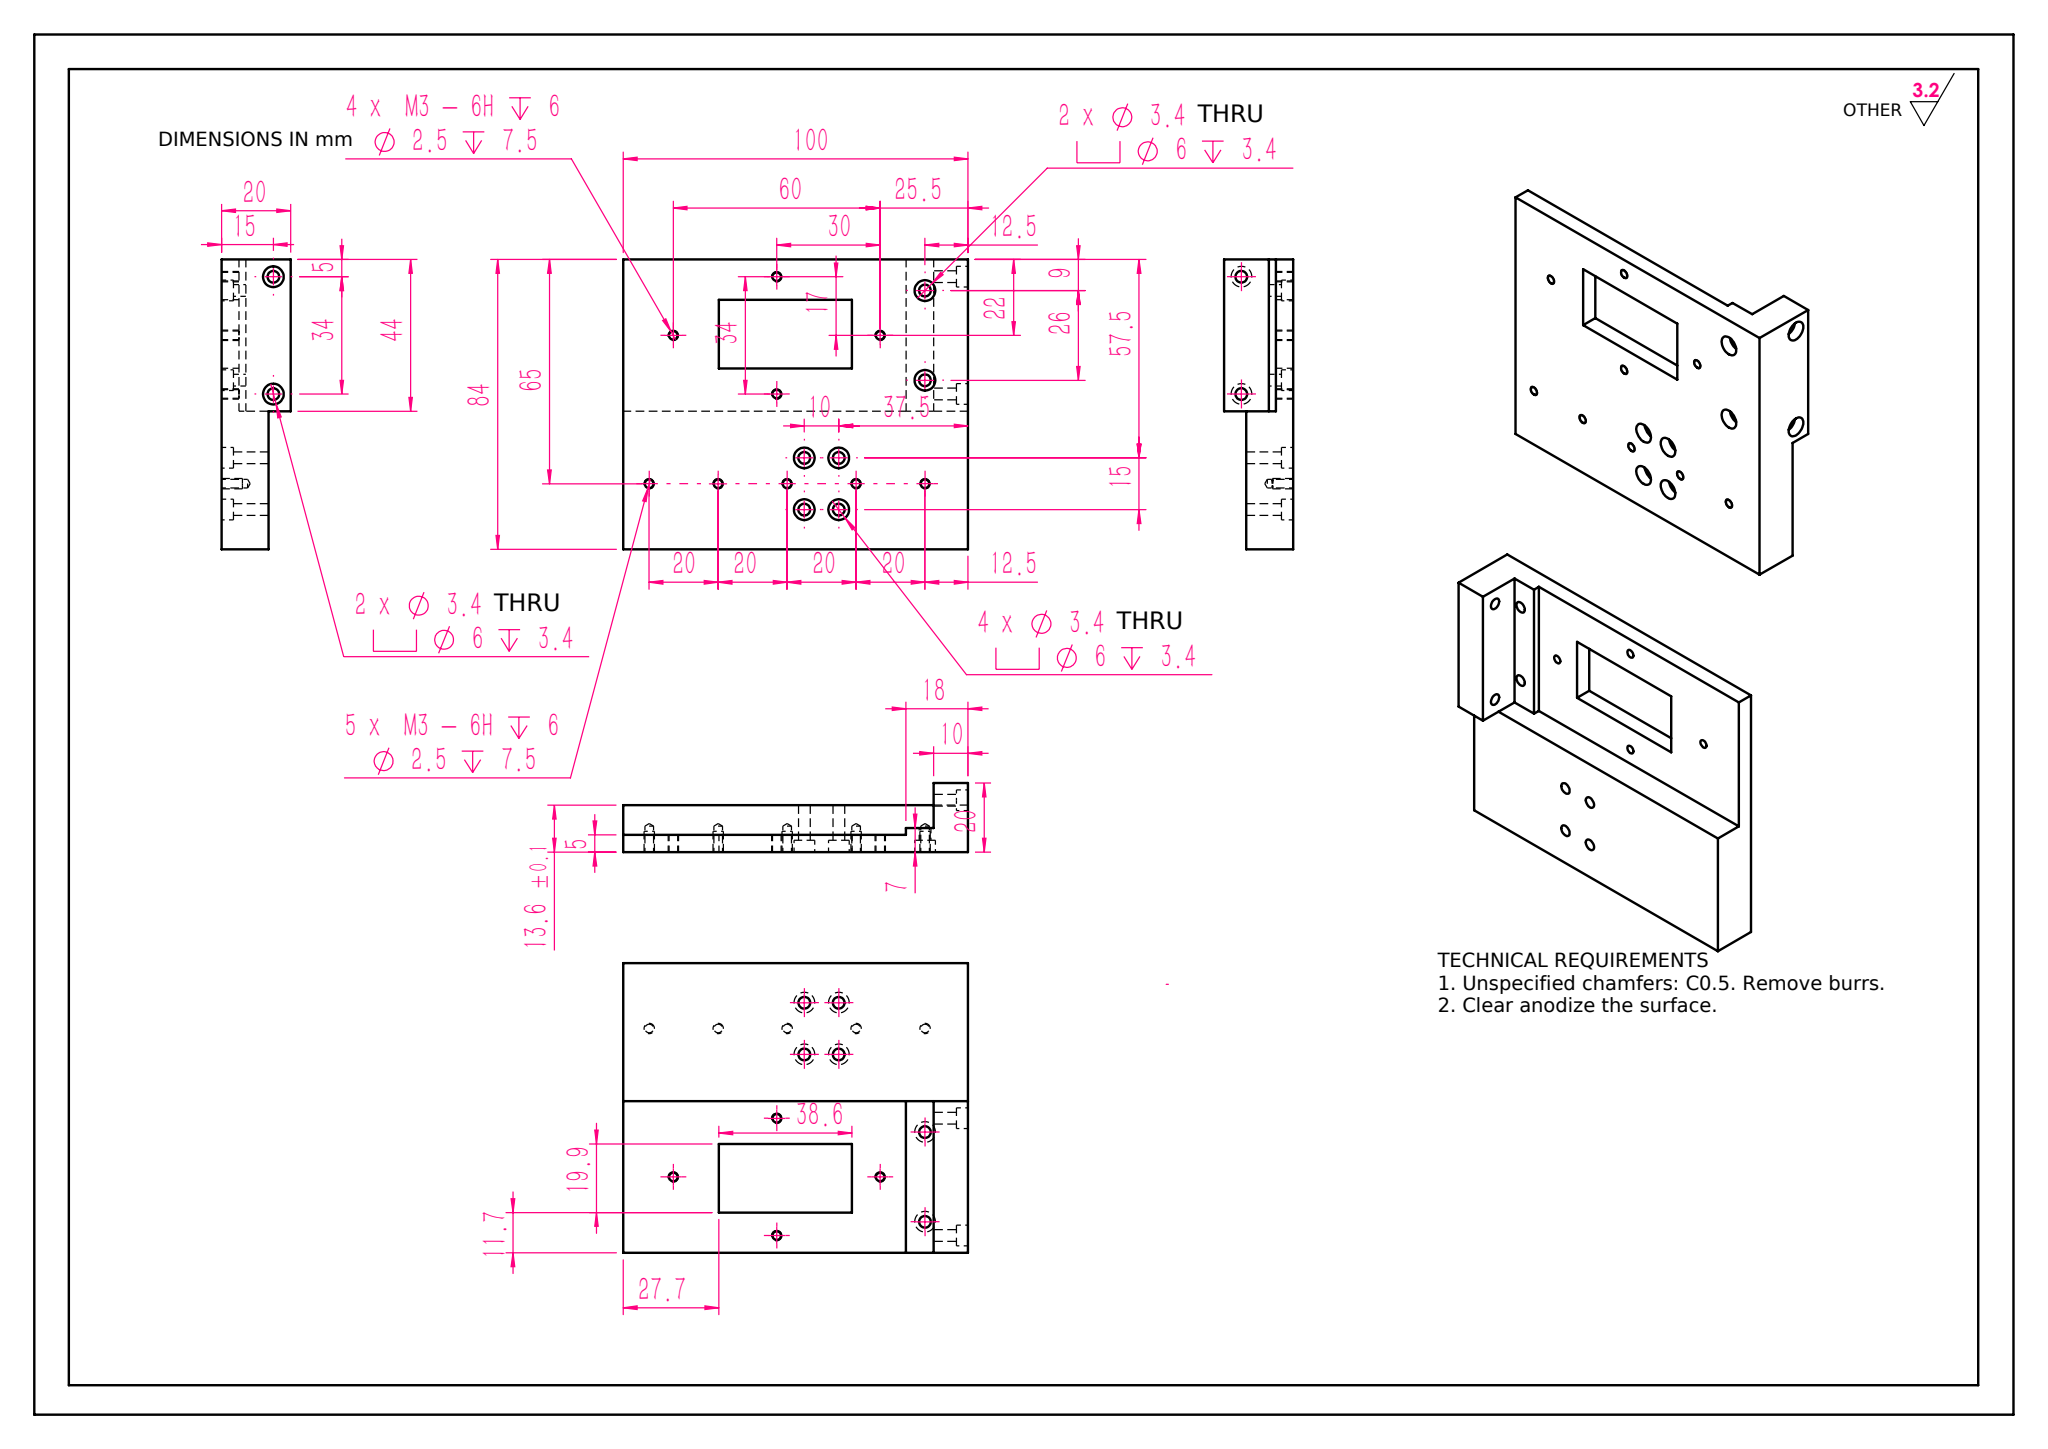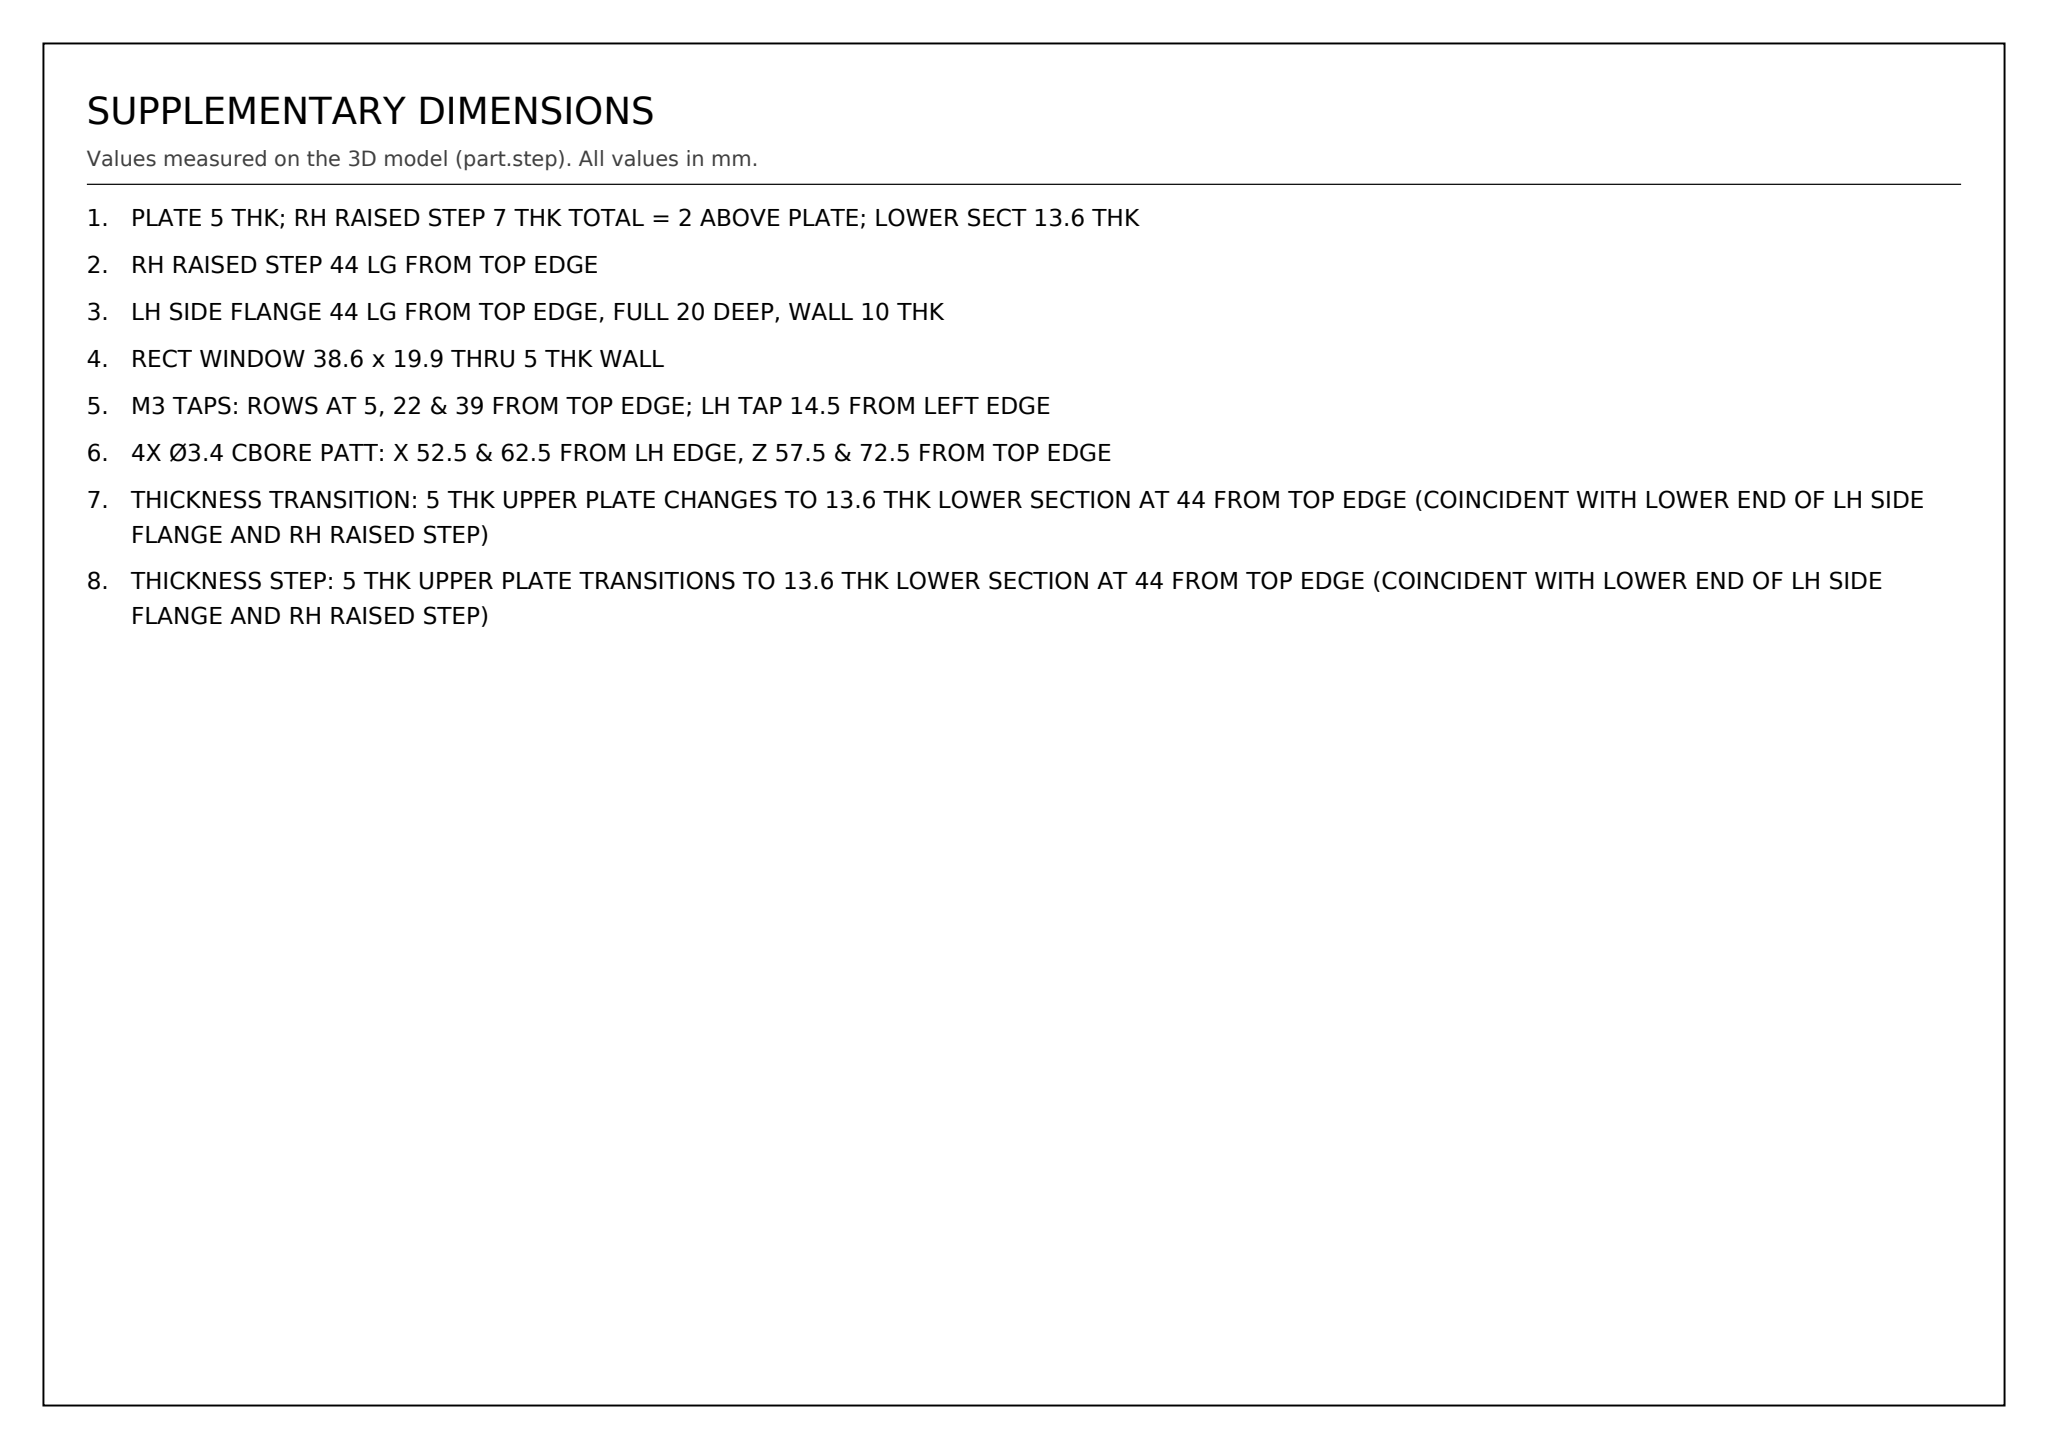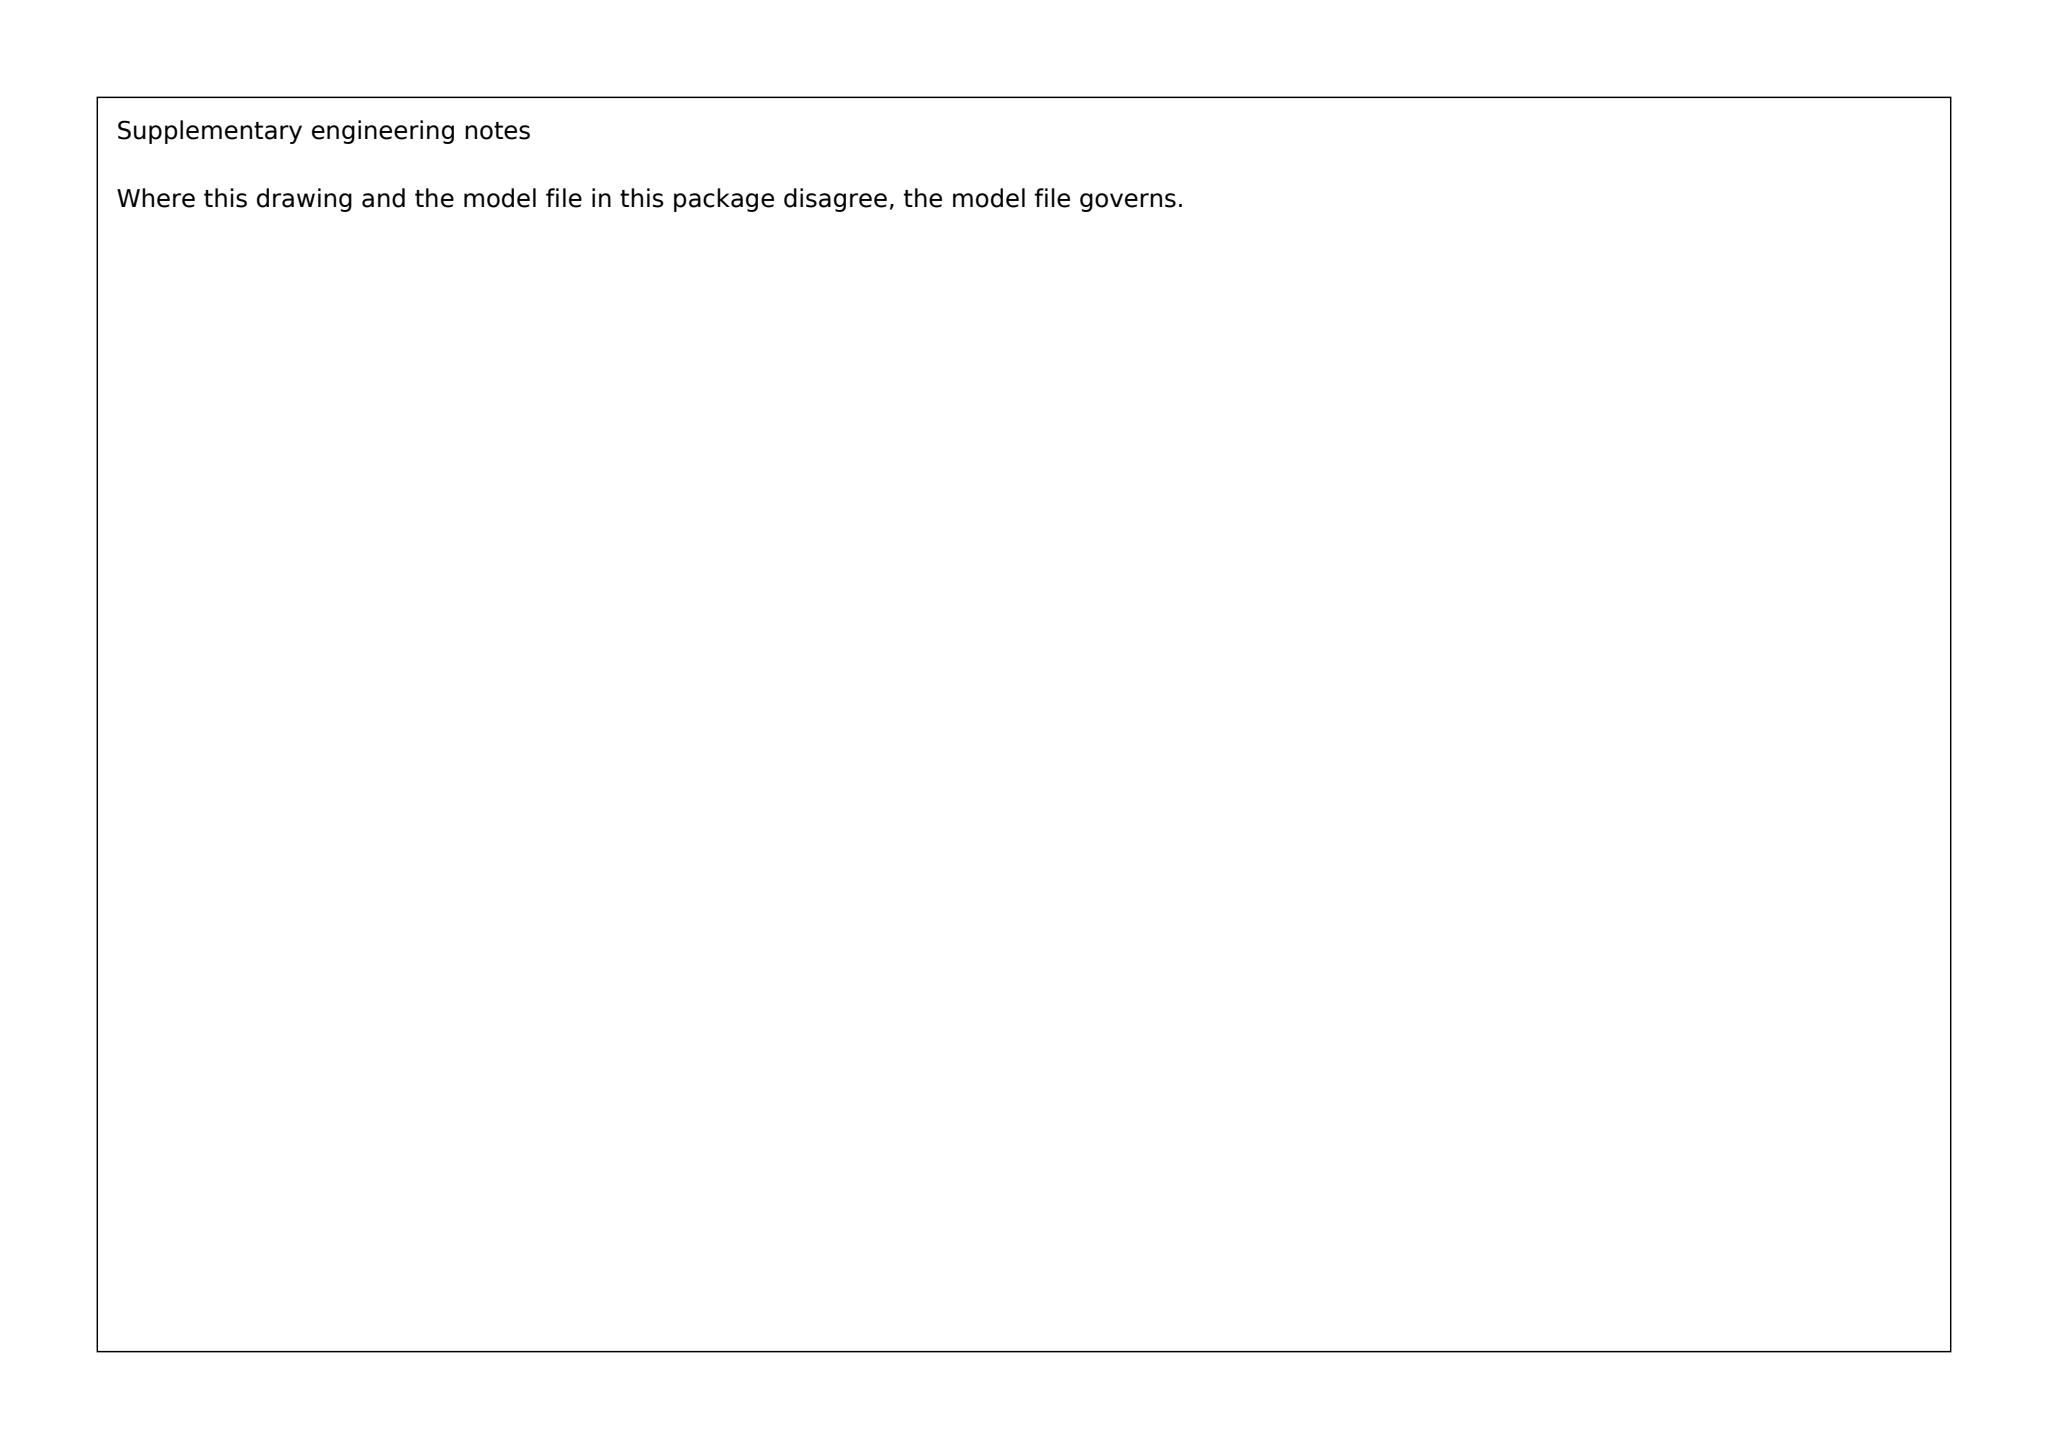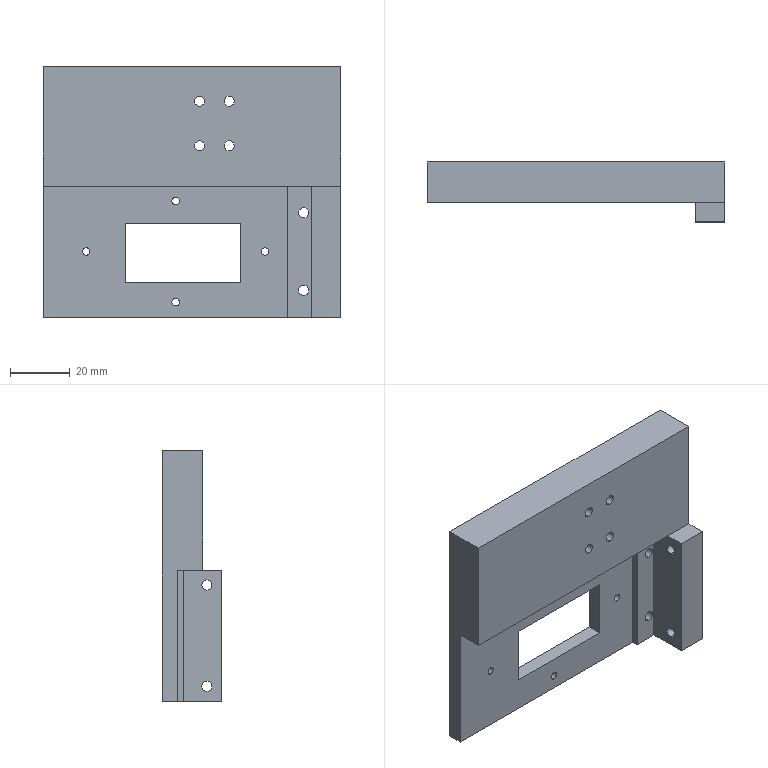Part | SolidWorks | mm | 1 solid | 85 faces | box 100 x 20 x 84 mm | volume 78254 mm3 | cylinder 50 | plane 25 | cone 10 | commonest cylinder face diameters 2.5 x18 6 x16 3.4 x16
Drawing notes:
PLATE 5 THK; RH RAISED STEP 7 THK TOTAL = 2 ABOVE PLATE; LOWER SECT 13.6 THK | from the solid: y-planes 13 & 15 vs face y=20: 20-13=7 step, 20-15=5 plate, diff 2; lower zone y=6.4 (13.6)
RH RAISED STEP 44 LG FROM TOP EDGE | from the solid: step faces x=82/90, y=13; z plane at 44.0 ends step
LH SIDE FLANGE 44 LG FROM TOP EDGE, FULL 20 DEEP, WALL 10 THK | from the solid: z-planes 0 & 44 bound flange; bbox y=20 depth; O3.4 thru 6.6 + O6 cbore 3.4 = 10 wall
RECT WINDOW 38.6 x 19.9 THRU 5 THK WALL | from the solid: X 27.72/66.34 (38.62), Z 11.68/31.55 (19.87); no intermediate Y plane 15.0-20.0 -> thru
M3 TAPS: ROWS AT 5, 22 & 39 FROM TOP EDGE; LH TAP 14.5 FROM LEFT EDGE | from the solid: M3 cyls z=5 (x44.5), z=22 (x14.5 & 74.5), z=39 (x44.5); 17 & 34 chain, 60 chain in X
4X Ø3.4 CBORE PATT: X 52.5 & 62.5 FROM LH EDGE, Z 57.5 & 72.5 FROM TOP EDGE | from the solid: O3.4/O6 cbore axes y at x=52.5/62.5 (10 apart), z=57.5/72.5 (15 apart)
THICKNESS TRANSITION: 5 THK UPPER PLATE CHANGES TO 13.6 THK LOWER SECTION AT 44 FROM TOP EDGE (COINCIDENT WITH LOWER END OF LH SIDE FLANGE AND RH RAISED STEP) | from the solid: Supplementary dims 1, 2 & 3: PLATE 5 THK, LOWER SECT 13.6 THK; RH RAISED STEP 44 LG FROM TOP EDGE; LH SIDE FLANGE 44 LG FROM TOP EDGE
THICKNESS STEP: 5 THK UPPER PLATE TRANSITIONS TO 13.6 THK LOWER SECTION AT 44 FROM TOP EDGE (COINCIDENT WITH LOWER END OF LH SIDE FLANGE AND RH RAISED STEP) | from the solid: Supplementary dimension 7: thickness transition 5 THK to 13.6 THK at 44 from top edge, coincident with lower end of LH side flange and RH raised step
build123d program:
from build123d import *

# Parameters (mm, degrees)
SKETCH1_W                                            = 100
SKETCH1_H                                            = 44
BOSS_EXTRUDE1_DEPTH                                  = 20
SKETCH2_W                                            = 90
SKETCH2_H                                            = 13
CUT_EXTRUDE1_DEPTH                                   = 70.541
SKETCH3_W                                            = 82
SKETCH3_H                                            = 2
CUT_EXTRUDE2_DEPTH                                   = 70.541
HOLE_SIZE_ACCORDING_TO_THE_TYPE_OF_HEXAG_D           = 3.4
HOLE_SIZE_ACCORDING_TO_THE_TYPE_OF_HEXAG_CBORE_D     = 6
HOLE_SIZE_ACCORDING_TO_THE_TYPE_OF_HEXAG_CBORE_DEPTH = 3.4
HOLE_SIZE_ACCORDING_TO_THE_TYPE_OF_H_2_D             = 3.4
HOLE_SIZE_ACCORDING_TO_THE_TYPE_OF_H_2_CBORE_D       = 6
HOLE_SIZE_ACCORDING_TO_THE_TYPE_OF_H_2_CBORE_DEPTH   = 3.4
M3_TAPPED_HOLE1_D                                    = 2.5
M3_TAPPED_HOLE1_DEPTH                                = 7.5
M3_TAPPED_HOLE1_TIP                                  = 0.7511
BOSS_EXTRUDE2_START                                  = -44
SKETCH11_W                                           = 100
SKETCH11_H                                           = 13.6
BOSS_EXTRUDE2_DEPTH                                  = 40
HOLE_SIZE_ACCORDING_TO_THE_TYPE_OF_H_3_D             = 3.4
HOLE_SIZE_ACCORDING_TO_THE_TYPE_OF_H_3_CBORE_D       = 6
HOLE_SIZE_ACCORDING_TO_THE_TYPE_OF_H_3_CBORE_DEPTH   = 3.4
LPATTERN1_COUNT                                      = 5
LPATTERN1_PITCH                                      = 20
SKETCH20_W                                           = 38.621
SKETCH20_H                                           = 19.87
CUT_EXTRUDE3_DEPTH                                   = 125


with BuildPart() as part:
    # Sketch1 → Boss-Extrude1 (new body)
    with BuildSketch(Plane(origin=(0, 0, 0), x_dir=(1, 0, 0), z_dir=(0, 1, 0))):
        Rectangle(SKETCH1_W, SKETCH1_H)
    extrude(amount=BOSS_EXTRUDE1_DEPTH)

    # Sketch2 → Cut-Extrude1 (cut, through all)
    with BuildSketch(Plane(origin=(0, 0, -22), x_dir=(-1, 0, 0), z_dir=(0, 0, -1))):
        with Locations((5, 6.5)):
            Rectangle(SKETCH2_W, SKETCH2_H)
    extrude(amount=-CUT_EXTRUDE1_DEPTH, mode=Mode.SUBTRACT)

    # Sketch3 → Cut-Extrude2 (cut, through all)
    with BuildSketch(Plane(origin=(0, 0, -22), x_dir=(-1, 0, 0), z_dir=(0, 0, -1))):
        with Locations((9, 14)):
            Rectangle(SKETCH3_W, SKETCH3_H)
    extrude(amount=-CUT_EXTRUDE2_DEPTH, mode=Mode.SUBTRACT)

    # Hole Size according to the type of Hexag (through all)
    with Locations(Plane(origin=(50, 0, 0), x_dir=(0, 0, -1), z_dir=(1, 0, 0))):
        with Locations((-17, 5), (17, 5)):
            CounterBoreHole(HOLE_SIZE_ACCORDING_TO_THE_TYPE_OF_HEXAG_D / 2, HOLE_SIZE_ACCORDING_TO_THE_TYPE_OF_HEXAG_CBORE_D / 2, HOLE_SIZE_ACCORDING_TO_THE_TYPE_OF_HEXAG_CBORE_DEPTH)

    # Hole Size according to the type of H 2 (through all)
    with Locations(Plane(origin=(0, 20, 0), x_dir=(1, 0, 0), z_dir=(0, 1, 0))):
        with Locations((37.5, 13), (37.5, -13)):
            CounterBoreHole(HOLE_SIZE_ACCORDING_TO_THE_TYPE_OF_H_2_D / 2, HOLE_SIZE_ACCORDING_TO_THE_TYPE_OF_H_2_CBORE_D / 2, HOLE_SIZE_ACCORDING_TO_THE_TYPE_OF_H_2_CBORE_DEPTH)

    # M3 Tapped Hole1
    with Locations(Plane(origin=(0, 20, 0), x_dir=(1, 0, 0), z_dir=(0, 1, 0))):
        with Locations((24.5, 0), (-5.5, -17), (-5.5, 17), (-35.5, 0)):
            Hole(M3_TAPPED_HOLE1_D / 2, depth=M3_TAPPED_HOLE1_DEPTH)
            with Locations((0, 0, -(M3_TAPPED_HOLE1_DEPTH + M3_TAPPED_HOLE1_TIP / 2))):  # 118° drill point
                Cone(0, M3_TAPPED_HOLE1_D / 2, M3_TAPPED_HOLE1_TIP, mode=Mode.SUBTRACT)

    # Sketch11 → Boss-Extrude2 (add)
    with BuildSketch(Plane(origin=(0, 0, -22), x_dir=(-1, 0, 0), z_dir=(0, 0, -1)).offset(BOSS_EXTRUDE2_START)):
        with Locations((0, 13.2)):
            Rectangle(SKETCH11_W, SKETCH11_H)
    extrude(amount=-BOSS_EXTRUDE2_DEPTH)

    # Hole Size according to the type of H 3 (through all)
    with Locations(Plane(origin=(0, 20, 0), x_dir=(1, 0, 0), z_dir=(0, 1, 0))):
        with Locations((12.5, -50.5), (12.5, -35.5), (2.5, -50.5), (2.5, -35.5)):
            CounterBoreHole(HOLE_SIZE_ACCORDING_TO_THE_TYPE_OF_H_3_D / 2, HOLE_SIZE_ACCORDING_TO_THE_TYPE_OF_H_3_CBORE_D / 2, HOLE_SIZE_ACCORDING_TO_THE_TYPE_OF_H_3_CBORE_DEPTH)

    # Sketch18 → M3 Tapped Hole2 (revolve, cut)
    with BuildSketch(Plane(origin=(-42.5, 20, 43), x_dir=(0, 0, 1), z_dir=(1, 0, 0))):
        Polygon((0, 0), (0, 8.251), (1.25, 7.5), (1.25, 0), align=None)
    m3_tapped_hole2 = revolve(axis=Axis((-42.5, 26.35, 43), (0, -1, 0)), mode=Mode.SUBTRACT)

    # LPattern1: M3 Tapped Hole2 ×5
    with Locations(*[(i * LPATTERN1_PITCH, 0, 0) for i in range(1, LPATTERN1_COUNT)]):
        add(m3_tapped_hole2, mode=Mode.SUBTRACT)

    # Sketch20 → Cut-Extrude3 (cut)
    with BuildSketch(Plane.XZ.offset(-15)):
        with Locations((-2.968, -0.3859)):
            Rectangle(SKETCH20_W, SKETCH20_H)
    extrude(amount=-CUT_EXTRUDE3_DEPTH, mode=Mode.SUBTRACT)


solid = part.part